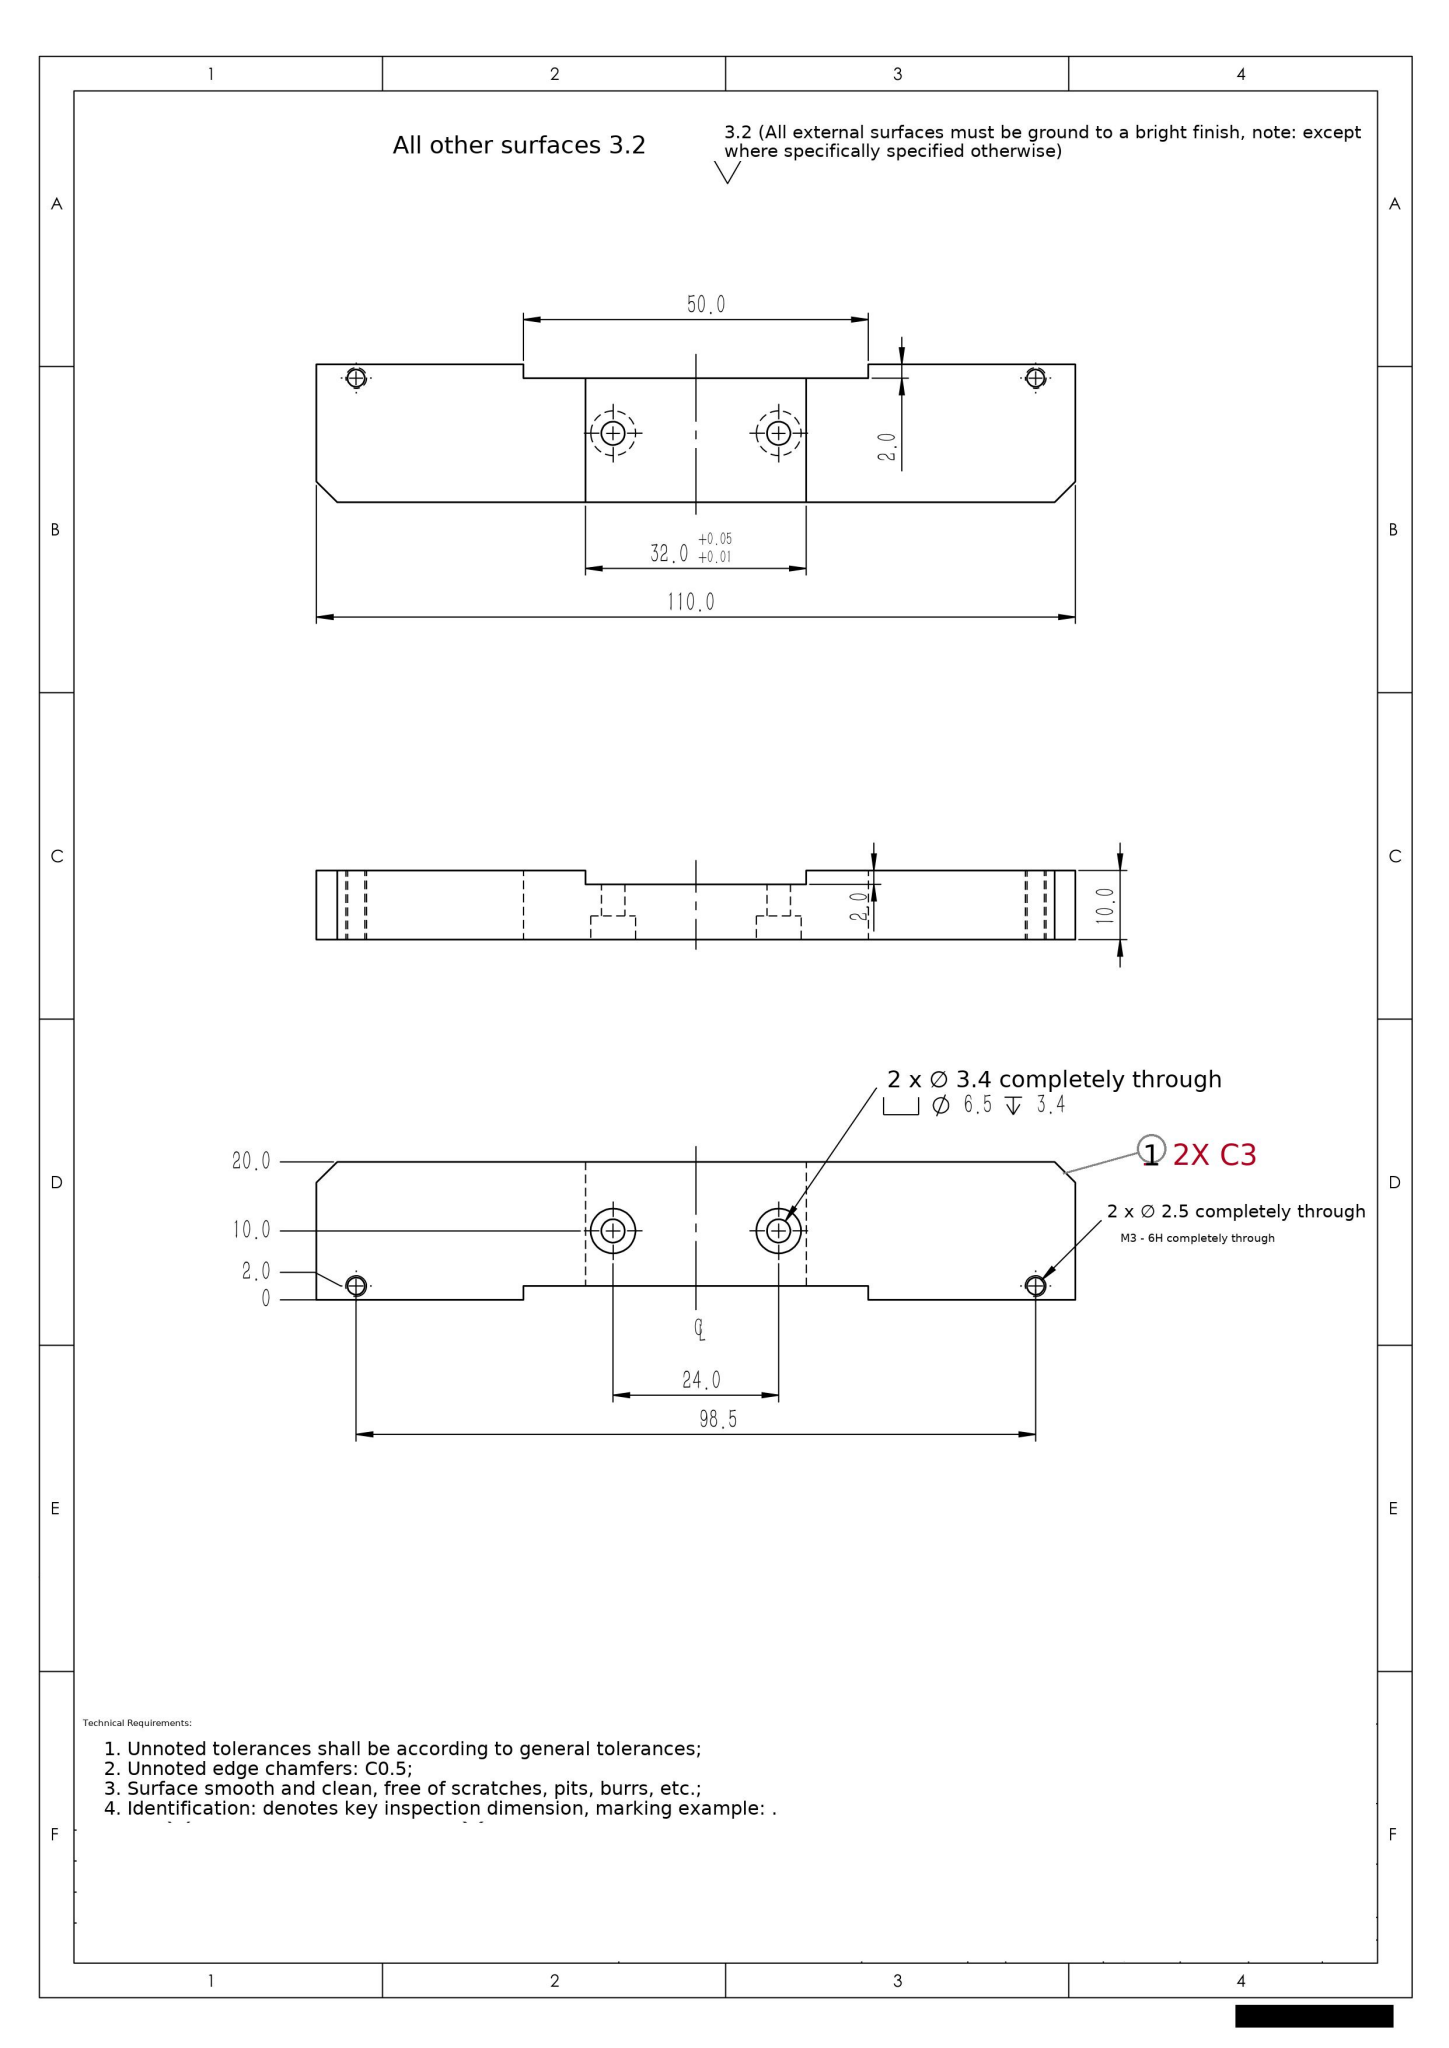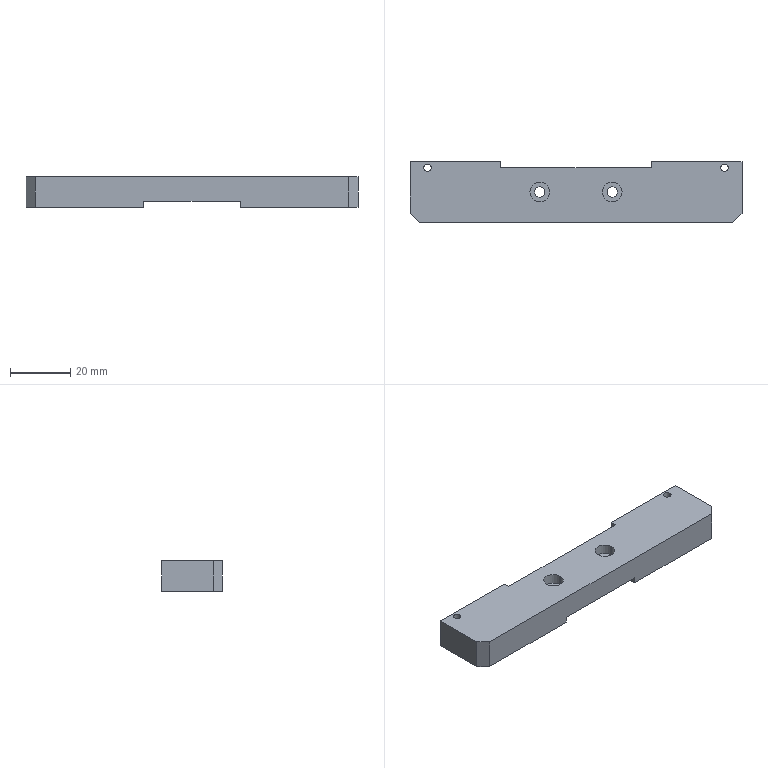Part | SolidWorks | mm | 1 solid | 30 faces | box 110 x 20 x 10 mm | volume 19351 mm3 | plane 18 | cylinder 12 | commonest cylinder face diameters 6.5 x4 3.4 x4 2.5 x4
build123d program:
from build123d import *

# Parameters (mm, degrees)
SKETCH1_W                                       = 110
SKETCH1_H                                       = 20
BOSS_EXTRUDE1_DEPTH                             = 5
M3_TAPPED_HOLE1_D                               = 2.5
M3_HEX_SOCKET_HEAD_CAP_SCREW_CBORE1_D           = 3.4
M3_HEX_SOCKET_HEAD_CAP_SCREW_CBORE1_CBORE_D     = 6.5
M3_HEX_SOCKET_HEAD_CAP_SCREW_CBORE1_CBORE_DEPTH = 3.4
SKETCH17_W                                      = 32
SKETCH17_H                                      = 18.5
CUT_EXTRUDE2_DEPTH                              = 2
SKETCH18_W                                      = 50
SKETCH18_H                                      = 2
CUT_EXTRUDE3_DEPTH                              = 57.789
CHAMFER1_SIZE                                   = 3


with BuildPart() as part:
    # Sketch1 → Boss-Extrude1 (new, symmetric)
    with BuildSketch(Plane.XY):
        Rectangle(SKETCH1_W, SKETCH1_H)
    extrude(amount=BOSS_EXTRUDE1_DEPTH, both=True)

    # M3 Tapped Hole1 (through all)
    with Locations(Plane.XY.offset(5)):
        with Locations((-49.25, 8), (49.25, 8)):
            Hole(M3_TAPPED_HOLE1_D / 2)

    # M3 Hex Socket Head Cap Screw CBORE1 (through all)
    with Locations(Plane.XY.offset(5)):
        with Locations((-12, 0), (12, 0)):
            CounterBoreHole(M3_HEX_SOCKET_HEAD_CAP_SCREW_CBORE1_D / 2, M3_HEX_SOCKET_HEAD_CAP_SCREW_CBORE1_CBORE_D / 2, M3_HEX_SOCKET_HEAD_CAP_SCREW_CBORE1_CBORE_DEPTH)

    # Sketch17 → Cut-Extrude2 (cut)
    with BuildSketch(Plane(origin=(0, 0, -5), x_dir=(-1, 0, 0), z_dir=(0, 0, -1))):
        with Locations((0, -0.75)):
            Rectangle(SKETCH17_W, SKETCH17_H)
    extrude(amount=-CUT_EXTRUDE2_DEPTH, mode=Mode.SUBTRACT)

    # Sketch18 → Cut-Extrude3 (cut, through all)
    with BuildSketch(Plane(origin=(0, 0, -5), x_dir=(-1, 0, 0), z_dir=(0, 0, -1))):
        with Locations((0, 9)):
            Rectangle(SKETCH18_W, SKETCH18_H)
    extrude(amount=-CUT_EXTRUDE3_DEPTH, mode=Mode.SUBTRACT)

    # Chamfer1
    chamfer1_edges = [part.edges().sort_by_distance(p)[0] for p in [
        (55, -10, 0),
        (-55, -10, 0),
    ]]
    chamfer(chamfer1_edges, length=CHAMFER1_SIZE)


solid = part.part
STEP:
#1=CARTESIAN_POINT('',(-15.25,0.,1.6));
#2=VERTEX_POINT('',#1);
#3=CARTESIAN_POINT('',(-8.75,0.,1.6));
#4=VERTEX_POINT('',#3);
#5=CARTESIAN_POINT('',(-12.,0.,1.6));
#6=DIRECTION('',(0.,0.,1.));
#7=DIRECTION('',(1.,0.,0.));
#8=AXIS2_PLACEMENT_3D('',#5,#6,#7);
#9=CIRCLE('',#8,3.25);
#10=EDGE_CURVE('',#2,#4,#9,.T.);
#11=ORIENTED_EDGE('',*,*,#10,.F.);
#12=CARTESIAN_POINT('',(-15.25,0.,5.));
#13=VERTEX_POINT('',#12);
#14=CARTESIAN_POINT('',(-15.25,0.,5.));
#15=DIRECTION('',(0.,0.,1.));
#16=VECTOR('',#15,1000.);
#17=LINE('',#14,#16);
#18=EDGE_CURVE('',#2,#13,#17,.T.);
#19=ORIENTED_EDGE('',*,*,#18,.T.);
#20=CARTESIAN_POINT('',(-8.75,0.,5.));
#21=VERTEX_POINT('',#20);
#22=CARTESIAN_POINT('',(-12.,0.,5.));
#23=DIRECTION('',(0.,0.,1.));
#24=DIRECTION('',(1.,0.,0.));
#25=AXIS2_PLACEMENT_3D('',#22,#23,#24);
#26=CIRCLE('',#25,3.25);
#27=EDGE_CURVE('',#13,#21,#26,.T.);
#28=ORIENTED_EDGE('',*,*,#27,.T.);
#29=CARTESIAN_POINT('',(-8.75,0.,5.));
#30=DIRECTION('',(0.,0.,1.));
#31=VECTOR('',#30,1000.);
#32=LINE('',#29,#31);
#33=EDGE_CURVE('',#4,#21,#32,.T.);
#34=ORIENTED_EDGE('',*,*,#33,.F.);
#35=EDGE_LOOP('',(#11,#19,#28,#34));
#36=FACE_OUTER_BOUND('',#35,.T.);
#37=CARTESIAN_POINT('',(-12.,0.,5.));
#38=DIRECTION('',(0.,0.,1.));
#39=DIRECTION('',(1.,0.,0.));
#40=AXIS2_PLACEMENT_3D('',#37,#38,#39);
#41=CYLINDRICAL_SURFACE('',#40,3.25);
#42=ADVANCED_FACE('',(#36),#41,.F.);
#43=CARTESIAN_POINT('',(-10.3,0.,-3.));
#44=VERTEX_POINT('',#43);
#45=CARTESIAN_POINT('',(-13.7,0.,-3.));
#46=VERTEX_POINT('',#45);
#47=CARTESIAN_POINT('',(-12.,0.,-3.));
#48=DIRECTION('',(0.,0.,-1.));
#49=DIRECTION('',(1.,0.,0.));
#50=AXIS2_PLACEMENT_3D('',#47,#48,#49);
#51=CIRCLE('',#50,1.7);
#52=EDGE_CURVE('',#44,#46,#51,.T.);
#53=ORIENTED_EDGE('',*,*,#52,.T.);
#54=CARTESIAN_POINT('',(-13.7,0.,1.6));
#55=VERTEX_POINT('',#54);
#56=CARTESIAN_POINT('',(-13.7,0.,5.));
#57=DIRECTION('',(0.,0.,1.));
#58=VECTOR('',#57,1000.);
#59=LINE('',#56,#58);
#60=EDGE_CURVE('',#46,#55,#59,.T.);
#61=ORIENTED_EDGE('',*,*,#60,.T.);
#62=CARTESIAN_POINT('',(-10.3,0.,1.6));
#63=VERTEX_POINT('',#62);
#64=CARTESIAN_POINT('',(-12.,0.,1.6));
#65=DIRECTION('',(0.,0.,1.));
#66=DIRECTION('',(1.,0.,0.));
#67=AXIS2_PLACEMENT_3D('',#64,#65,#66);
#68=CIRCLE('',#67,1.7);
#69=EDGE_CURVE('',#55,#63,#68,.T.);
#70=ORIENTED_EDGE('',*,*,#69,.T.);
#71=CARTESIAN_POINT('',(-10.3,0.,5.));
#72=DIRECTION('',(0.,0.,1.));
#73=VECTOR('',#72,1000.);
#74=LINE('',#71,#73);
#75=EDGE_CURVE('',#44,#63,#74,.T.);
#76=ORIENTED_EDGE('',*,*,#75,.F.);
#77=EDGE_LOOP('',(#53,#61,#70,#76));
#78=FACE_OUTER_BOUND('',#77,.T.);
#79=CARTESIAN_POINT('',(-12.,0.,5.));
#80=DIRECTION('',(0.,0.,1.));
#81=DIRECTION('',(1.,0.,0.));
#82=AXIS2_PLACEMENT_3D('',#79,#80,#81);
#83=CYLINDRICAL_SURFACE('',#82,1.7);
#84=ADVANCED_FACE('',(#78),#83,.F.);
#85=CARTESIAN_POINT('',(8.75,0.,1.6));
#86=VERTEX_POINT('',#85);
#87=CARTESIAN_POINT('',(15.25,0.,1.6));
#88=VERTEX_POINT('',#87);
#89=CARTESIAN_POINT('',(12.,0.,1.6));
#90=DIRECTION('',(0.,0.,1.));
#91=DIRECTION('',(1.,0.,0.));
#92=AXIS2_PLACEMENT_3D('',#89,#90,#91);
#93=CIRCLE('',#92,3.25);
#94=EDGE_CURVE('',#86,#88,#93,.T.);
#95=ORIENTED_EDGE('',*,*,#94,.F.);
#96=CARTESIAN_POINT('',(8.75,0.,5.));
#97=VERTEX_POINT('',#96);
#98=CARTESIAN_POINT('',(8.75,0.,5.));
#99=DIRECTION('',(0.,0.,1.));
#100=VECTOR('',#99,1000.);
#101=LINE('',#98,#100);
#102=EDGE_CURVE('',#86,#97,#101,.T.);
#103=ORIENTED_EDGE('',*,*,#102,.T.);
#104=CARTESIAN_POINT('',(15.25,0.,5.));
#105=VERTEX_POINT('',#104);
#106=CARTESIAN_POINT('',(12.,0.,5.));
#107=DIRECTION('',(0.,0.,1.));
#108=DIRECTION('',(1.,0.,0.));
#109=AXIS2_PLACEMENT_3D('',#106,#107,#108);
#110=CIRCLE('',#109,3.25);
#111=EDGE_CURVE('',#97,#105,#110,.T.);
#112=ORIENTED_EDGE('',*,*,#111,.T.);
#113=CARTESIAN_POINT('',(15.25,0.,5.));
#114=DIRECTION('',(0.,0.,1.));
#115=VECTOR('',#114,1000.);
#116=LINE('',#113,#115);
#117=EDGE_CURVE('',#88,#105,#116,.T.);
#118=ORIENTED_EDGE('',*,*,#117,.F.);
#119=EDGE_LOOP('',(#95,#103,#112,#118));
#120=FACE_OUTER_BOUND('',#119,.T.);
#121=CARTESIAN_POINT('',(12.,0.,5.));
#122=DIRECTION('',(0.,0.,1.));
#123=DIRECTION('',(1.,0.,0.));
#124=AXIS2_PLACEMENT_3D('',#121,#122,#123);
#125=CYLINDRICAL_SURFACE('',#124,3.25);
#126=ADVANCED_FACE('',(#120),#125,.F.);
#127=CARTESIAN_POINT('',(13.7,0.,-3.));
#128=VERTEX_POINT('',#127);
#129=CARTESIAN_POINT('',(10.3,0.,-3.));
#130=VERTEX_POINT('',#129);
#131=CARTESIAN_POINT('',(12.,0.,-3.));
#132=DIRECTION('',(0.,0.,-1.));
#133=DIRECTION('',(1.,0.,0.));
#134=AXIS2_PLACEMENT_3D('',#131,#132,#133);
#135=CIRCLE('',#134,1.7);
#136=EDGE_CURVE('',#128,#130,#135,.T.);
#137=ORIENTED_EDGE('',*,*,#136,.T.);
#138=CARTESIAN_POINT('',(10.3,0.,1.6));
#139=VERTEX_POINT('',#138);
#140=CARTESIAN_POINT('',(10.3,0.,5.));
#141=DIRECTION('',(0.,0.,1.));
#142=VECTOR('',#141,1000.);
#143=LINE('',#140,#142);
#144=EDGE_CURVE('',#130,#139,#143,.T.);
#145=ORIENTED_EDGE('',*,*,#144,.T.);
#146=CARTESIAN_POINT('',(13.7,0.,1.6));
#147=VERTEX_POINT('',#146);
#148=CARTESIAN_POINT('',(12.,0.,1.6));
#149=DIRECTION('',(0.,0.,1.));
#150=DIRECTION('',(1.,0.,0.));
#151=AXIS2_PLACEMENT_3D('',#148,#149,#150);
#152=CIRCLE('',#151,1.7);
#153=EDGE_CURVE('',#139,#147,#152,.T.);
#154=ORIENTED_EDGE('',*,*,#153,.T.);
#155=CARTESIAN_POINT('',(13.7,0.,5.));
#156=DIRECTION('',(0.,0.,1.));
#157=VECTOR('',#156,1000.);
#158=LINE('',#155,#157);
#159=EDGE_CURVE('',#128,#147,#158,.T.);
#160=ORIENTED_EDGE('',*,*,#159,.F.);
#161=EDGE_LOOP('',(#137,#145,#154,#160));
#162=FACE_OUTER_BOUND('',#161,.T.);
#163=CARTESIAN_POINT('',(12.,0.,5.));
#164=DIRECTION('',(0.,0.,1.));
#165=DIRECTION('',(1.,0.,0.));
#166=AXIS2_PLACEMENT_3D('',#163,#164,#165);
#167=CYLINDRICAL_SURFACE('',#166,1.7);
#168=ADVANCED_FACE('',(#162),#167,.F.);
#169=CARTESIAN_POINT('',(-50.5,8.,-5.));
#170=VERTEX_POINT('',#169);
#171=CARTESIAN_POINT('',(-48.,8.,-5.));
#172=VERTEX_POINT('',#171);
#173=CARTESIAN_POINT('',(-49.25,8.,-5.));
#174=DIRECTION('',(0.,0.,1.));
#175=DIRECTION('',(1.,0.,0.));
#176=AXIS2_PLACEMENT_3D('',#173,#174,#175);
#177=CIRCLE('',#176,1.25);
#178=EDGE_CURVE('',#170,#172,#177,.T.);
#179=ORIENTED_EDGE('',*,*,#178,.F.);
#180=CARTESIAN_POINT('',(-50.5,8.,5.));
#181=VERTEX_POINT('',#180);
#182=CARTESIAN_POINT('',(-50.5,8.,5.));
#183=DIRECTION('',(0.,0.,1.));
#184=VECTOR('',#183,1000.);
#185=LINE('',#182,#184);
#186=EDGE_CURVE('',#170,#181,#185,.T.);
#187=ORIENTED_EDGE('',*,*,#186,.T.);
#188=CARTESIAN_POINT('',(-48.,8.,5.));
#189=VERTEX_POINT('',#188);
#190=CARTESIAN_POINT('',(-49.25,8.,5.));
#191=DIRECTION('',(0.,0.,1.));
#192=DIRECTION('',(1.,0.,0.));
#193=AXIS2_PLACEMENT_3D('',#190,#191,#192);
#194=CIRCLE('',#193,1.25);
#195=EDGE_CURVE('',#181,#189,#194,.T.);
#196=ORIENTED_EDGE('',*,*,#195,.T.);
#197=CARTESIAN_POINT('',(-48.,8.,5.));
#198=DIRECTION('',(0.,0.,1.));
#199=VECTOR('',#198,1000.);
#200=LINE('',#197,#199);
#201=EDGE_CURVE('',#172,#189,#200,.T.);
#202=ORIENTED_EDGE('',*,*,#201,.F.);
#203=EDGE_LOOP('',(#179,#187,#196,#202));
#204=FACE_OUTER_BOUND('',#203,.T.);
#205=CARTESIAN_POINT('',(-49.25,8.,5.));
#206=DIRECTION('',(0.,0.,1.));
#207=DIRECTION('',(1.,0.,0.));
#208=AXIS2_PLACEMENT_3D('',#205,#206,#207);
#209=CYLINDRICAL_SURFACE('',#208,1.25);
#210=ADVANCED_FACE('',(#204),#209,.F.);
#211=CARTESIAN_POINT('',(48.,8.,-5.));
#212=VERTEX_POINT('',#211);
#213=CARTESIAN_POINT('',(50.5,8.,-5.));
#214=VERTEX_POINT('',#213);
#215=CARTESIAN_POINT('',(49.25,8.,-5.));
#216=DIRECTION('',(0.,0.,1.));
#217=DIRECTION('',(1.,0.,0.));
#218=AXIS2_PLACEMENT_3D('',#215,#216,#217);
#219=CIRCLE('',#218,1.25);
#220=EDGE_CURVE('',#212,#214,#219,.T.);
#221=ORIENTED_EDGE('',*,*,#220,.F.);
#222=CARTESIAN_POINT('',(48.,8.,5.));
#223=VERTEX_POINT('',#222);
#224=CARTESIAN_POINT('',(48.,8.,5.));
#225=DIRECTION('',(0.,0.,1.));
#226=VECTOR('',#225,1000.);
#227=LINE('',#224,#226);
#228=EDGE_CURVE('',#212,#223,#227,.T.);
#229=ORIENTED_EDGE('',*,*,#228,.T.);
#230=CARTESIAN_POINT('',(50.5,8.,5.));
#231=VERTEX_POINT('',#230);
#232=CARTESIAN_POINT('',(49.25,8.,5.));
#233=DIRECTION('',(0.,0.,1.));
#234=DIRECTION('',(1.,0.,0.));
#235=AXIS2_PLACEMENT_3D('',#232,#233,#234);
#236=CIRCLE('',#235,1.25);
#237=EDGE_CURVE('',#223,#231,#236,.T.);
#238=ORIENTED_EDGE('',*,*,#237,.T.);
#239=CARTESIAN_POINT('',(50.5,8.,5.));
#240=DIRECTION('',(0.,0.,1.));
#241=VECTOR('',#240,1000.);
#242=LINE('',#239,#241);
#243=EDGE_CURVE('',#214,#231,#242,.T.);
#244=ORIENTED_EDGE('',*,*,#243,.F.);
#245=EDGE_LOOP('',(#221,#229,#238,#244));
#246=FACE_OUTER_BOUND('',#245,.T.);
#247=CARTESIAN_POINT('',(49.25,8.,5.));
#248=DIRECTION('',(0.,0.,1.));
#249=DIRECTION('',(1.,0.,0.));
#250=AXIS2_PLACEMENT_3D('',#247,#248,#249);
#251=CYLINDRICAL_SURFACE('',#250,1.25);
#252=ADVANCED_FACE('',(#246),#251,.F.);
#253=CARTESIAN_POINT('',(-25.,10.,5.));
#254=VERTEX_POINT('',#253);
#255=CARTESIAN_POINT('',(-55.,10.,5.));
#256=VERTEX_POINT('',#255);
#257=CARTESIAN_POINT('',(-55.,10.,5.));
#258=DIRECTION('',(-1.,0.,0.));
#259=VECTOR('',#258,1000.);
#260=LINE('',#257,#259);
#261=EDGE_CURVE('',#254,#256,#260,.T.);
#262=ORIENTED_EDGE('',*,*,#261,.F.);
#263=CARTESIAN_POINT('',(-25.,10.,-5.));
#264=VERTEX_POINT('',#263);
#265=CARTESIAN_POINT('',(-25.,10.,5.));
#266=DIRECTION('',(0.,0.,-1.));
#267=VECTOR('',#266,1000.);
#268=LINE('',#265,#267);
#269=EDGE_CURVE('',#254,#264,#268,.T.);
#270=ORIENTED_EDGE('',*,*,#269,.T.);
#271=CARTESIAN_POINT('',(-55.,10.,-5.));
#272=VERTEX_POINT('',#271);
#273=CARTESIAN_POINT('',(-55.,10.,-5.));
#274=DIRECTION('',(-1.,0.,0.));
#275=VECTOR('',#274,1000.);
#276=LINE('',#273,#275);
#277=EDGE_CURVE('',#264,#272,#276,.T.);
#278=ORIENTED_EDGE('',*,*,#277,.T.);
#279=CARTESIAN_POINT('',(-55.,10.,5.));
#280=DIRECTION('',(0.,0.,-1.));
#281=VECTOR('',#280,1000.);
#282=LINE('',#279,#281);
#283=EDGE_CURVE('',#256,#272,#282,.T.);
#284=ORIENTED_EDGE('',*,*,#283,.F.);
#285=EDGE_LOOP('',(#262,#270,#278,#284));
#286=FACE_OUTER_BOUND('',#285,.T.);
#287=CARTESIAN_POINT('',(-55.,10.,5.));
#288=DIRECTION('',(0.,-1.,0.));
#289=DIRECTION('',(0.,0.,-1.));
#290=AXIS2_PLACEMENT_3D('',#287,#288,#289);
#291=PLANE('',#290);
#292=ADVANCED_FACE('',(#286),#291,.F.);
#293=CARTESIAN_POINT('',(-52.,-10.,-5.));
#294=VERTEX_POINT('',#293);
#295=CARTESIAN_POINT('',(-16.,-10.,-5.));
#296=VERTEX_POINT('',#295);
#297=CARTESIAN_POINT('',(-55.,-10.,-5.));
#298=DIRECTION('',(1.,0.,0.));
#299=VECTOR('',#298,1000.);
#300=LINE('',#297,#299);
#301=EDGE_CURVE('',#294,#296,#300,.T.);
#302=ORIENTED_EDGE('',*,*,#301,.F.);
#303=CARTESIAN_POINT('',(-55.,-7.,-5.));
#304=VERTEX_POINT('',#303);
#305=CARTESIAN_POINT('',(-31.,-31.,-5.));
#306=DIRECTION('',(-0.7071,0.7071,0.));
#307=VECTOR('',#306,1000.);
#308=LINE('',#305,#307);
#309=EDGE_CURVE('',#294,#304,#308,.T.);
#310=ORIENTED_EDGE('',*,*,#309,.T.);
#311=CARTESIAN_POINT('',(-55.,-10.,-5.));
#312=DIRECTION('',(0.,-1.,0.));
#313=VECTOR('',#312,1000.);
#314=LINE('',#311,#313);
#315=EDGE_CURVE('',#272,#304,#314,.T.);
#316=ORIENTED_EDGE('',*,*,#315,.F.);
#317=ORIENTED_EDGE('',*,*,#277,.F.);
#318=CARTESIAN_POINT('',(-25.,8.,-5.));
#319=VERTEX_POINT('',#318);
#320=CARTESIAN_POINT('',(-25.,10.,-5.));
#321=DIRECTION('',(-0.,1.,0.));
#322=VECTOR('',#321,1000.);
#323=LINE('',#320,#322);
#324=EDGE_CURVE('',#319,#264,#323,.T.);
#325=ORIENTED_EDGE('',*,*,#324,.F.);
#326=CARTESIAN_POINT('',(-16.,8.,-5.));
#327=VERTEX_POINT('',#326);
#328=CARTESIAN_POINT('',(-25.,8.,-5.));
#329=DIRECTION('',(-1.,-0.,0.));
#330=VECTOR('',#329,1000.);
#331=LINE('',#328,#330);
#332=EDGE_CURVE('',#327,#319,#331,.T.);
#333=ORIENTED_EDGE('',*,*,#332,.F.);
#334=CARTESIAN_POINT('',(-16.,8.5,-5.));
#335=DIRECTION('',(0.,1.,0.));
#336=VECTOR('',#335,1000.);
#337=LINE('',#334,#336);
#338=EDGE_CURVE('',#296,#327,#337,.T.);
#339=ORIENTED_EDGE('',*,*,#338,.F.);
#340=EDGE_LOOP('',(#302,#310,#316,#317,#325,#333,#339));
#341=FACE_OUTER_BOUND('',#340,.T.);
#342=CARTESIAN_POINT('',(-49.25,8.,-5.));
#343=DIRECTION('',(0.,0.,1.));
#344=DIRECTION('',(1.,0.,0.));
#345=AXIS2_PLACEMENT_3D('',#342,#343,#344);
#346=CIRCLE('',#345,1.25);
#347=EDGE_CURVE('',#172,#170,#346,.T.);
#348=ORIENTED_EDGE('',*,*,#347,.T.);
#349=ORIENTED_EDGE('',*,*,#178,.T.);
#350=EDGE_LOOP('',(#348,#349));
#351=FACE_BOUND('',#350,.T.);
#352=CARTESIAN_POINT('',(0.,0.,-5.));
#353=DIRECTION('',(0.,0.,-1.));
#354=DIRECTION('',(-1.,0.,0.));
#355=AXIS2_PLACEMENT_3D('',#352,#353,#354);
#356=PLANE('',#355);
#357=ADVANCED_FACE('',(#341,#351),#356,.T.);
#358=CARTESIAN_POINT('',(55.,-7.,5.));
#359=VERTEX_POINT('',#358);
#360=CARTESIAN_POINT('',(55.,10.,5.));
#361=VERTEX_POINT('',#360);
#362=CARTESIAN_POINT('',(55.,-10.,5.));
#363=DIRECTION('',(0.,1.,0.));
#364=VECTOR('',#363,1000.);
#365=LINE('',#362,#364);
#366=EDGE_CURVE('',#359,#361,#365,.T.);
#367=ORIENTED_EDGE('',*,*,#366,.F.);
#368=CARTESIAN_POINT('',(55.,-7.,-5.));
#369=VERTEX_POINT('',#368);
#370=CARTESIAN_POINT('',(55.,-7.,5.));
#371=DIRECTION('',(0.,0.,-1.));
#372=VECTOR('',#371,1000.);
#373=LINE('',#370,#372);
#374=EDGE_CURVE('',#359,#369,#373,.T.);
#375=ORIENTED_EDGE('',*,*,#374,.T.);
#376=CARTESIAN_POINT('',(55.,10.,-5.));
#377=VERTEX_POINT('',#376);
#378=CARTESIAN_POINT('',(55.,-10.,-5.));
#379=DIRECTION('',(0.,1.,0.));
#380=VECTOR('',#379,1000.);
#381=LINE('',#378,#380);
#382=EDGE_CURVE('',#369,#377,#381,.T.);
#383=ORIENTED_EDGE('',*,*,#382,.T.);
#384=CARTESIAN_POINT('',(55.,10.,5.));
#385=DIRECTION('',(0.,0.,-1.));
#386=VECTOR('',#385,1000.);
#387=LINE('',#384,#386);
#388=EDGE_CURVE('',#361,#377,#387,.T.);
#389=ORIENTED_EDGE('',*,*,#388,.F.);
#390=EDGE_LOOP('',(#367,#375,#383,#389));
#391=FACE_OUTER_BOUND('',#390,.T.);
#392=CARTESIAN_POINT('',(55.,-10.,5.));
#393=DIRECTION('',(-1.,0.,0.));
#394=DIRECTION('',(0.,0.,1.));
#395=AXIS2_PLACEMENT_3D('',#392,#393,#394);
#396=PLANE('',#395);
#397=ADVANCED_FACE('',(#391),#396,.F.);
#398=CARTESIAN_POINT('',(25.,10.,-5.));
#399=VERTEX_POINT('',#398);
#400=CARTESIAN_POINT('',(-55.,10.,-5.));
#401=DIRECTION('',(-1.,0.,0.));
#402=VECTOR('',#401,1000.);
#403=LINE('',#400,#402);
#404=EDGE_CURVE('',#377,#399,#403,.T.);
#405=ORIENTED_EDGE('',*,*,#404,.T.);
#406=CARTESIAN_POINT('',(25.,10.,5.));
#407=VERTEX_POINT('',#406);
#408=CARTESIAN_POINT('',(25.,10.,5.));
#409=DIRECTION('',(0.,0.,-1.));
#410=VECTOR('',#409,1000.);
#411=LINE('',#408,#410);
#412=EDGE_CURVE('',#407,#399,#411,.T.);
#413=ORIENTED_EDGE('',*,*,#412,.F.);
#414=CARTESIAN_POINT('',(-55.,10.,5.));
#415=DIRECTION('',(-1.,0.,0.));
#416=VECTOR('',#415,1000.);
#417=LINE('',#414,#416);
#418=EDGE_CURVE('',#361,#407,#417,.T.);
#419=ORIENTED_EDGE('',*,*,#418,.F.);
#420=ORIENTED_EDGE('',*,*,#388,.T.);
#421=EDGE_LOOP('',(#405,#413,#419,#420));
#422=FACE_OUTER_BOUND('',#421,.T.);
#423=CARTESIAN_POINT('',(-55.,10.,5.));
#424=DIRECTION('',(0.,-1.,0.));
#425=DIRECTION('',(0.,0.,-1.));
#426=AXIS2_PLACEMENT_3D('',#423,#424,#425);
#427=PLANE('',#426);
#428=ADVANCED_FACE('',(#422),#427,.F.);
#429=ORIENTED_EDGE('',*,*,#315,.T.);
#430=CARTESIAN_POINT('',(-55.,-7.,5.));
#431=VERTEX_POINT('',#430);
#432=CARTESIAN_POINT('',(-55.,-7.,5.));
#433=DIRECTION('',(0.,0.,1.));
#434=VECTOR('',#433,1000.);
#435=LINE('',#432,#434);
#436=EDGE_CURVE('',#304,#431,#435,.T.);
#437=ORIENTED_EDGE('',*,*,#436,.T.);
#438=CARTESIAN_POINT('',(-55.,-10.,5.));
#439=DIRECTION('',(0.,-1.,0.));
#440=VECTOR('',#439,1000.);
#441=LINE('',#438,#440);
#442=EDGE_CURVE('',#256,#431,#441,.T.);
#443=ORIENTED_EDGE('',*,*,#442,.F.);
#444=ORIENTED_EDGE('',*,*,#283,.T.);
#445=EDGE_LOOP('',(#429,#437,#443,#444));
#446=FACE_OUTER_BOUND('',#445,.T.);
#447=CARTESIAN_POINT('',(-55.,-10.,5.));
#448=DIRECTION('',(1.,0.,0.));
#449=DIRECTION('',(0.,0.,-1.));
#450=AXIS2_PLACEMENT_3D('',#447,#448,#449);
#451=PLANE('',#450);
#452=ADVANCED_FACE('',(#446),#451,.F.);
#453=CARTESIAN_POINT('',(16.,-10.,-5.));
#454=VERTEX_POINT('',#453);
#455=CARTESIAN_POINT('',(52.,-10.,-5.));
#456=VERTEX_POINT('',#455);
#457=CARTESIAN_POINT('',(-55.,-10.,-5.));
#458=DIRECTION('',(1.,0.,0.));
#459=VECTOR('',#458,1000.);
#460=LINE('',#457,#459);
#461=EDGE_CURVE('',#454,#456,#460,.T.);
#462=ORIENTED_EDGE('',*,*,#461,.T.);
#463=CARTESIAN_POINT('',(52.,-10.,5.));
#464=VERTEX_POINT('',#463);
#465=CARTESIAN_POINT('',(52.,-10.,5.));
#466=DIRECTION('',(0.,0.,1.));
#467=VECTOR('',#466,1000.);
#468=LINE('',#465,#467);
#469=EDGE_CURVE('',#456,#464,#468,.T.);
#470=ORIENTED_EDGE('',*,*,#469,.T.);
#471=CARTESIAN_POINT('',(-52.,-10.,5.));
#472=VERTEX_POINT('',#471);
#473=CARTESIAN_POINT('',(-55.,-10.,5.));
#474=DIRECTION('',(1.,0.,0.));
#475=VECTOR('',#474,1000.);
#476=LINE('',#473,#475);
#477=EDGE_CURVE('',#472,#464,#476,.T.);
#478=ORIENTED_EDGE('',*,*,#477,.F.);
#479=CARTESIAN_POINT('',(-52.,-10.,5.));
#480=DIRECTION('',(0.,0.,-1.));
#481=VECTOR('',#480,1000.);
#482=LINE('',#479,#481);
#483=EDGE_CURVE('',#472,#294,#482,.T.);
#484=ORIENTED_EDGE('',*,*,#483,.T.);
#485=ORIENTED_EDGE('',*,*,#301,.T.);
#486=CARTESIAN_POINT('',(-16.,-10.,-3.));
#487=VERTEX_POINT('',#486);
#488=CARTESIAN_POINT('',(-16.,-10.,-3.));
#489=DIRECTION('',(0.,0.,-1.));
#490=VECTOR('',#489,1000.);
#491=LINE('',#488,#490);
#492=EDGE_CURVE('',#487,#296,#491,.T.);
#493=ORIENTED_EDGE('',*,*,#492,.F.);
#494=CARTESIAN_POINT('',(16.,-10.,-3.));
#495=VERTEX_POINT('',#494);
#496=CARTESIAN_POINT('',(-16.,-10.,-3.));
#497=DIRECTION('',(-1.,-0.,0.));
#498=VECTOR('',#497,1000.);
#499=LINE('',#496,#498);
#500=EDGE_CURVE('',#495,#487,#499,.T.);
#501=ORIENTED_EDGE('',*,*,#500,.F.);
#502=CARTESIAN_POINT('',(16.,-10.,-3.));
#503=DIRECTION('',(0.,0.,-1.));
#504=VECTOR('',#503,1000.);
#505=LINE('',#502,#504);
#506=EDGE_CURVE('',#495,#454,#505,.T.);
#507=ORIENTED_EDGE('',*,*,#506,.T.);
#508=EDGE_LOOP('',(#462,#470,#478,#484,#485,#493,#501,#507));
#509=FACE_OUTER_BOUND('',#508,.T.);
#510=CARTESIAN_POINT('',(-55.,-10.,5.));
#511=DIRECTION('',(0.,1.,0.));
#512=DIRECTION('',(0.,0.,1.));
#513=AXIS2_PLACEMENT_3D('',#510,#511,#512);
#514=PLANE('',#513);
#515=ADVANCED_FACE('',(#509),#514,.F.);
#516=CARTESIAN_POINT('',(-12.,0.,5.));
#517=DIRECTION('',(0.,0.,1.));
#518=DIRECTION('',(1.,0.,0.));
#519=AXIS2_PLACEMENT_3D('',#516,#517,#518);
#520=CIRCLE('',#519,3.25);
#521=EDGE_CURVE('',#21,#13,#520,.T.);
#522=ORIENTED_EDGE('',*,*,#521,.F.);
#523=ORIENTED_EDGE('',*,*,#27,.F.);
#524=EDGE_LOOP('',(#522,#523));
#525=FACE_BOUND('',#524,.T.);
#526=CARTESIAN_POINT('',(12.,0.,5.));
#527=DIRECTION('',(0.,0.,1.));
#528=DIRECTION('',(1.,0.,0.));
#529=AXIS2_PLACEMENT_3D('',#526,#527,#528);
#530=CIRCLE('',#529,3.25);
#531=EDGE_CURVE('',#105,#97,#530,.T.);
#532=ORIENTED_EDGE('',*,*,#531,.F.);
#533=ORIENTED_EDGE('',*,*,#111,.F.);
#534=EDGE_LOOP('',(#532,#533));
#535=FACE_BOUND('',#534,.T.);
#536=CARTESIAN_POINT('',(-49.25,8.,5.));
#537=DIRECTION('',(0.,0.,1.));
#538=DIRECTION('',(1.,0.,0.));
#539=AXIS2_PLACEMENT_3D('',#536,#537,#538);
#540=CIRCLE('',#539,1.25);
#541=EDGE_CURVE('',#189,#181,#540,.T.);
#542=ORIENTED_EDGE('',*,*,#541,.F.);
#543=ORIENTED_EDGE('',*,*,#195,.F.);
#544=EDGE_LOOP('',(#542,#543));
#545=FACE_BOUND('',#544,.T.);
#546=CARTESIAN_POINT('',(49.25,8.,5.));
#547=DIRECTION('',(0.,0.,1.));
#548=DIRECTION('',(1.,0.,0.));
#549=AXIS2_PLACEMENT_3D('',#546,#547,#548);
#550=CIRCLE('',#549,1.25);
#551=EDGE_CURVE('',#231,#223,#550,.T.);
#552=ORIENTED_EDGE('',*,*,#551,.F.);
#553=ORIENTED_EDGE('',*,*,#237,.F.);
#554=EDGE_LOOP('',(#552,#553));
#555=FACE_BOUND('',#554,.T.);
#556=ORIENTED_EDGE('',*,*,#477,.T.);
#557=CARTESIAN_POINT('',(55.,-7.,5.));
#558=DIRECTION('',(0.7071,0.7071,0.));
#559=VECTOR('',#558,1000.);
#560=LINE('',#557,#559);
#561=EDGE_CURVE('',#464,#359,#560,.T.);
#562=ORIENTED_EDGE('',*,*,#561,.T.);
#563=ORIENTED_EDGE('',*,*,#366,.T.);
#564=ORIENTED_EDGE('',*,*,#418,.T.);
#565=CARTESIAN_POINT('',(25.,8.,5.));
#566=VERTEX_POINT('',#565);
#567=CARTESIAN_POINT('',(25.,10.,5.));
#568=DIRECTION('',(0.,-1.,0.));
#569=VECTOR('',#568,1000.);
#570=LINE('',#567,#569);
#571=EDGE_CURVE('',#407,#566,#570,.T.);
#572=ORIENTED_EDGE('',*,*,#571,.T.);
#573=CARTESIAN_POINT('',(-25.,8.,5.));
#574=VERTEX_POINT('',#573);
#575=CARTESIAN_POINT('',(-25.,8.,5.));
#576=DIRECTION('',(-1.,-0.,0.));
#577=VECTOR('',#576,1000.);
#578=LINE('',#575,#577);
#579=EDGE_CURVE('',#566,#574,#578,.T.);
#580=ORIENTED_EDGE('',*,*,#579,.T.);
#581=CARTESIAN_POINT('',(-25.,10.,5.));
#582=DIRECTION('',(-0.,1.,0.));
#583=VECTOR('',#582,1000.);
#584=LINE('',#581,#583);
#585=EDGE_CURVE('',#574,#254,#584,.T.);
#586=ORIENTED_EDGE('',*,*,#585,.T.);
#587=ORIENTED_EDGE('',*,*,#261,.T.);
#588=ORIENTED_EDGE('',*,*,#442,.T.);
#589=CARTESIAN_POINT('',(-52.,-10.,5.));
#590=DIRECTION('',(0.7071,-0.7071,0.));
#591=VECTOR('',#590,1000.);
#592=LINE('',#589,#591);
#593=EDGE_CURVE('',#431,#472,#592,.T.);
#594=ORIENTED_EDGE('',*,*,#593,.T.);
#595=EDGE_LOOP('',(#556,#562,#563,#564,#572,#580,#586,#587,#588,#594));
#596=FACE_OUTER_BOUND('',#595,.T.);
#597=CARTESIAN_POINT('',(0.,0.,5.));
#598=DIRECTION('',(0.,0.,-1.));
#599=DIRECTION('',(-1.,0.,0.));
#600=AXIS2_PLACEMENT_3D('',#597,#598,#599);
#601=PLANE('',#600);
#602=ADVANCED_FACE('',(#525,#535,#545,#555,#596),#601,.F.);
#603=ORIENTED_EDGE('',*,*,#382,.F.);
#604=CARTESIAN_POINT('',(31.,-31.,-5.));
#605=DIRECTION('',(-0.7071,-0.7071,0.));
#606=VECTOR('',#605,1000.);
#607=LINE('',#604,#606);
#608=EDGE_CURVE('',#369,#456,#607,.T.);
#609=ORIENTED_EDGE('',*,*,#608,.T.);
#610=ORIENTED_EDGE('',*,*,#461,.F.);
#611=CARTESIAN_POINT('',(16.,8.,-5.));
#612=VERTEX_POINT('',#611);
#613=CARTESIAN_POINT('',(16.,8.5,-5.));
#614=DIRECTION('',(0.,-1.,0.));
#615=VECTOR('',#614,1000.);
#616=LINE('',#613,#615);
#617=EDGE_CURVE('',#612,#454,#616,.T.);
#618=ORIENTED_EDGE('',*,*,#617,.F.);
#619=CARTESIAN_POINT('',(25.,8.,-5.));
#620=VERTEX_POINT('',#619);
#621=CARTESIAN_POINT('',(-25.,8.,-5.));
#622=DIRECTION('',(-1.,-0.,0.));
#623=VECTOR('',#622,1000.);
#624=LINE('',#621,#623);
#625=EDGE_CURVE('',#620,#612,#624,.T.);
#626=ORIENTED_EDGE('',*,*,#625,.F.);
#627=CARTESIAN_POINT('',(25.,10.,-5.));
#628=DIRECTION('',(0.,-1.,0.));
#629=VECTOR('',#628,1000.);
#630=LINE('',#627,#629);
#631=EDGE_CURVE('',#399,#620,#630,.T.);
#632=ORIENTED_EDGE('',*,*,#631,.F.);
#633=ORIENTED_EDGE('',*,*,#404,.F.);
#634=EDGE_LOOP('',(#603,#609,#610,#618,#626,#632,#633));
#635=FACE_OUTER_BOUND('',#634,.T.);
#636=CARTESIAN_POINT('',(49.25,8.,-5.));
#637=DIRECTION('',(0.,0.,1.));
#638=DIRECTION('',(1.,0.,0.));
#639=AXIS2_PLACEMENT_3D('',#636,#637,#638);
#640=CIRCLE('',#639,1.25);
#641=EDGE_CURVE('',#214,#212,#640,.T.);
#642=ORIENTED_EDGE('',*,*,#641,.T.);
#643=ORIENTED_EDGE('',*,*,#220,.T.);
#644=EDGE_LOOP('',(#642,#643));
#645=FACE_BOUND('',#644,.T.);
#646=CARTESIAN_POINT('',(0.,0.,-5.));
#647=DIRECTION('',(0.,0.,-1.));
#648=DIRECTION('',(-1.,0.,0.));
#649=AXIS2_PLACEMENT_3D('',#646,#647,#648);
#650=PLANE('',#649);
#651=ADVANCED_FACE('',(#635,#645),#650,.T.);
#652=ORIENTED_EDGE('',*,*,#228,.F.);
#653=ORIENTED_EDGE('',*,*,#641,.F.);
#654=ORIENTED_EDGE('',*,*,#243,.T.);
#655=ORIENTED_EDGE('',*,*,#551,.T.);
#656=EDGE_LOOP('',(#652,#653,#654,#655));
#657=FACE_OUTER_BOUND('',#656,.T.);
#658=CARTESIAN_POINT('',(49.25,8.,5.));
#659=DIRECTION('',(0.,0.,1.));
#660=DIRECTION('',(1.,0.,0.));
#661=AXIS2_PLACEMENT_3D('',#658,#659,#660);
#662=CYLINDRICAL_SURFACE('',#661,1.25);
#663=ADVANCED_FACE('',(#657),#662,.F.);
#664=ORIENTED_EDGE('',*,*,#186,.F.);
#665=ORIENTED_EDGE('',*,*,#347,.F.);
#666=ORIENTED_EDGE('',*,*,#201,.T.);
#667=ORIENTED_EDGE('',*,*,#541,.T.);
#668=EDGE_LOOP('',(#664,#665,#666,#667));
#669=FACE_OUTER_BOUND('',#668,.T.);
#670=CARTESIAN_POINT('',(-49.25,8.,5.));
#671=DIRECTION('',(0.,0.,1.));
#672=DIRECTION('',(1.,0.,0.));
#673=AXIS2_PLACEMENT_3D('',#670,#671,#672);
#674=CYLINDRICAL_SURFACE('',#673,1.25);
#675=ADVANCED_FACE('',(#669),#674,.F.);
#676=ORIENTED_EDGE('',*,*,#144,.F.);
#677=CARTESIAN_POINT('',(12.,0.,-3.));
#678=DIRECTION('',(0.,0.,-1.));
#679=DIRECTION('',(1.,0.,0.));
#680=AXIS2_PLACEMENT_3D('',#677,#678,#679);
#681=CIRCLE('',#680,1.7);
#682=EDGE_CURVE('',#130,#128,#681,.T.);
#683=ORIENTED_EDGE('',*,*,#682,.T.);
#684=ORIENTED_EDGE('',*,*,#159,.T.);
#685=CARTESIAN_POINT('',(12.,0.,1.6));
#686=DIRECTION('',(0.,0.,1.));
#687=DIRECTION('',(1.,0.,0.));
#688=AXIS2_PLACEMENT_3D('',#685,#686,#687);
#689=CIRCLE('',#688,1.7);
#690=EDGE_CURVE('',#147,#139,#689,.T.);
#691=ORIENTED_EDGE('',*,*,#690,.T.);
#692=EDGE_LOOP('',(#676,#683,#684,#691));
#693=FACE_OUTER_BOUND('',#692,.T.);
#694=CARTESIAN_POINT('',(12.,0.,5.));
#695=DIRECTION('',(0.,0.,1.));
#696=DIRECTION('',(1.,0.,0.));
#697=AXIS2_PLACEMENT_3D('',#694,#695,#696);
#698=CYLINDRICAL_SURFACE('',#697,1.7);
#699=ADVANCED_FACE('',(#693),#698,.F.);
#700=ORIENTED_EDGE('',*,*,#690,.F.);
#701=ORIENTED_EDGE('',*,*,#153,.F.);
#702=EDGE_LOOP('',(#700,#701));
#703=FACE_BOUND('',#702,.T.);
#704=CARTESIAN_POINT('',(12.,0.,1.6));
#705=DIRECTION('',(0.,0.,1.));
#706=DIRECTION('',(1.,0.,0.));
#707=AXIS2_PLACEMENT_3D('',#704,#705,#706);
#708=CIRCLE('',#707,3.25);
#709=EDGE_CURVE('',#88,#86,#708,.T.);
#710=ORIENTED_EDGE('',*,*,#709,.T.);
#711=ORIENTED_EDGE('',*,*,#94,.T.);
#712=EDGE_LOOP('',(#710,#711));
#713=FACE_OUTER_BOUND('',#712,.T.);
#714=CARTESIAN_POINT('',(13.7,0.,1.6));
#715=DIRECTION('',(0.,0.,-1.));
#716=DIRECTION('',(-1.,0.,0.));
#717=AXIS2_PLACEMENT_3D('',#714,#715,#716);
#718=PLANE('',#717);
#719=ADVANCED_FACE('',(#703,#713),#718,.F.);
#720=ORIENTED_EDGE('',*,*,#102,.F.);
#721=ORIENTED_EDGE('',*,*,#709,.F.);
#722=ORIENTED_EDGE('',*,*,#117,.T.);
#723=ORIENTED_EDGE('',*,*,#531,.T.);
#724=EDGE_LOOP('',(#720,#721,#722,#723));
#725=FACE_OUTER_BOUND('',#724,.T.);
#726=CARTESIAN_POINT('',(12.,0.,5.));
#727=DIRECTION('',(0.,0.,1.));
#728=DIRECTION('',(1.,0.,0.));
#729=AXIS2_PLACEMENT_3D('',#726,#727,#728);
#730=CYLINDRICAL_SURFACE('',#729,3.25);
#731=ADVANCED_FACE('',(#725),#730,.F.);
#732=ORIENTED_EDGE('',*,*,#60,.F.);
#733=CARTESIAN_POINT('',(-12.,0.,-3.));
#734=DIRECTION('',(0.,0.,-1.));
#735=DIRECTION('',(1.,0.,0.));
#736=AXIS2_PLACEMENT_3D('',#733,#734,#735);
#737=CIRCLE('',#736,1.7);
#738=EDGE_CURVE('',#46,#44,#737,.T.);
#739=ORIENTED_EDGE('',*,*,#738,.T.);
#740=ORIENTED_EDGE('',*,*,#75,.T.);
#741=CARTESIAN_POINT('',(-12.,0.,1.6));
#742=DIRECTION('',(0.,0.,1.));
#743=DIRECTION('',(1.,0.,0.));
#744=AXIS2_PLACEMENT_3D('',#741,#742,#743);
#745=CIRCLE('',#744,1.7);
#746=EDGE_CURVE('',#63,#55,#745,.T.);
#747=ORIENTED_EDGE('',*,*,#746,.T.);
#748=EDGE_LOOP('',(#732,#739,#740,#747));
#749=FACE_OUTER_BOUND('',#748,.T.);
#750=CARTESIAN_POINT('',(-12.,0.,5.));
#751=DIRECTION('',(0.,0.,1.));
#752=DIRECTION('',(1.,0.,0.));
#753=AXIS2_PLACEMENT_3D('',#750,#751,#752);
#754=CYLINDRICAL_SURFACE('',#753,1.7);
#755=ADVANCED_FACE('',(#749),#754,.F.);
#756=ORIENTED_EDGE('',*,*,#746,.F.);
#757=ORIENTED_EDGE('',*,*,#69,.F.);
#758=EDGE_LOOP('',(#756,#757));
#759=FACE_BOUND('',#758,.T.);
#760=CARTESIAN_POINT('',(-12.,0.,1.6));
#761=DIRECTION('',(0.,0.,1.));
#762=DIRECTION('',(1.,0.,0.));
#763=AXIS2_PLACEMENT_3D('',#760,#761,#762);
#764=CIRCLE('',#763,3.25);
#765=EDGE_CURVE('',#4,#2,#764,.T.);
#766=ORIENTED_EDGE('',*,*,#765,.T.);
#767=ORIENTED_EDGE('',*,*,#10,.T.);
#768=EDGE_LOOP('',(#766,#767));
#769=FACE_OUTER_BOUND('',#768,.T.);
#770=CARTESIAN_POINT('',(-10.3,0.,1.6));
#771=DIRECTION('',(0.,0.,-1.));
#772=DIRECTION('',(-1.,0.,0.));
#773=AXIS2_PLACEMENT_3D('',#770,#771,#772);
#774=PLANE('',#773);
#775=ADVANCED_FACE('',(#759,#769),#774,.F.);
#776=ORIENTED_EDGE('',*,*,#18,.F.);
#777=ORIENTED_EDGE('',*,*,#765,.F.);
#778=ORIENTED_EDGE('',*,*,#33,.T.);
#779=ORIENTED_EDGE('',*,*,#521,.T.);
#780=EDGE_LOOP('',(#776,#777,#778,#779));
#781=FACE_OUTER_BOUND('',#780,.T.);
#782=CARTESIAN_POINT('',(-12.,0.,5.));
#783=DIRECTION('',(0.,0.,1.));
#784=DIRECTION('',(1.,0.,0.));
#785=AXIS2_PLACEMENT_3D('',#782,#783,#784);
#786=CYLINDRICAL_SURFACE('',#785,3.25);
#787=ADVANCED_FACE('',(#781),#786,.F.);
#788=ORIENTED_EDGE('',*,*,#52,.F.);
#789=ORIENTED_EDGE('',*,*,#738,.F.);
#790=EDGE_LOOP('',(#788,#789));
#791=FACE_BOUND('',#790,.T.);
#792=CARTESIAN_POINT('',(-16.,8.,-3.));
#793=VERTEX_POINT('',#792);
#794=CARTESIAN_POINT('',(-16.,8.5,-3.));
#795=DIRECTION('',(0.,1.,0.));
#796=VECTOR('',#795,1000.);
#797=LINE('',#794,#796);
#798=EDGE_CURVE('',#487,#793,#797,.T.);
#799=ORIENTED_EDGE('',*,*,#798,.T.);
#800=CARTESIAN_POINT('',(16.,8.,-3.));
#801=VERTEX_POINT('',#800);
#802=CARTESIAN_POINT('',(-0.,8.,-3.));
#803=DIRECTION('',(1.,0.,0.));
#804=VECTOR('',#803,1000.);
#805=LINE('',#802,#804);
#806=EDGE_CURVE('',#793,#801,#805,.T.);
#807=ORIENTED_EDGE('',*,*,#806,.T.);
#808=CARTESIAN_POINT('',(16.,8.5,-3.));
#809=DIRECTION('',(0.,-1.,0.));
#810=VECTOR('',#809,1000.);
#811=LINE('',#808,#810);
#812=EDGE_CURVE('',#801,#495,#811,.T.);
#813=ORIENTED_EDGE('',*,*,#812,.T.);
#814=ORIENTED_EDGE('',*,*,#500,.T.);
#815=EDGE_LOOP('',(#799,#807,#813,#814));
#816=FACE_OUTER_BOUND('',#815,.T.);
#817=ORIENTED_EDGE('',*,*,#136,.F.);
#818=ORIENTED_EDGE('',*,*,#682,.F.);
#819=EDGE_LOOP('',(#817,#818));
#820=FACE_BOUND('',#819,.T.);
#821=CARTESIAN_POINT('',(0.,0.,-3.));
#822=DIRECTION('',(0.,0.,1.));
#823=DIRECTION('',(1.,0.,0.));
#824=AXIS2_PLACEMENT_3D('',#821,#822,#823);
#825=PLANE('',#824);
#826=ADVANCED_FACE('',(#791,#816,#820),#825,.F.);
#827=ORIENTED_EDGE('',*,*,#338,.T.);
#828=CARTESIAN_POINT('',(-16.,8.,-3.));
#829=DIRECTION('',(0.,0.,1.));
#830=VECTOR('',#829,1000.);
#831=LINE('',#828,#830);
#832=EDGE_CURVE('',#327,#793,#831,.T.);
#833=ORIENTED_EDGE('',*,*,#832,.T.);
#834=ORIENTED_EDGE('',*,*,#798,.F.);
#835=ORIENTED_EDGE('',*,*,#492,.T.);
#836=EDGE_LOOP('',(#827,#833,#834,#835));
#837=FACE_OUTER_BOUND('',#836,.T.);
#838=CARTESIAN_POINT('',(-16.,8.5,-3.));
#839=DIRECTION('',(-1.,0.,0.));
#840=DIRECTION('',(-0.,-1.,0.));
#841=AXIS2_PLACEMENT_3D('',#838,#839,#840);
#842=PLANE('',#841);
#843=ADVANCED_FACE('',(#837),#842,.F.);
#844=ORIENTED_EDGE('',*,*,#812,.F.);
#845=CARTESIAN_POINT('',(16.,8.,-3.));
#846=DIRECTION('',(0.,0.,-1.));
#847=VECTOR('',#846,1000.);
#848=LINE('',#845,#847);
#849=EDGE_CURVE('',#801,#612,#848,.T.);
#850=ORIENTED_EDGE('',*,*,#849,.T.);
#851=ORIENTED_EDGE('',*,*,#617,.T.);
#852=ORIENTED_EDGE('',*,*,#506,.F.);
#853=EDGE_LOOP('',(#844,#850,#851,#852));
#854=FACE_OUTER_BOUND('',#853,.T.);
#855=CARTESIAN_POINT('',(16.,8.5,-3.));
#856=DIRECTION('',(1.,0.,0.));
#857=DIRECTION('',(0.,0.,-1.));
#858=AXIS2_PLACEMENT_3D('',#855,#856,#857);
#859=PLANE('',#858);
#860=ADVANCED_FACE('',(#854),#859,.F.);
#861=ORIENTED_EDGE('',*,*,#332,.T.);
#862=CARTESIAN_POINT('',(-25.,8.,5.));
#863=DIRECTION('',(0.,0.,-1.));
#864=VECTOR('',#863,1000.);
#865=LINE('',#862,#864);
#866=EDGE_CURVE('',#574,#319,#865,.T.);
#867=ORIENTED_EDGE('',*,*,#866,.F.);
#868=ORIENTED_EDGE('',*,*,#579,.F.);
#869=CARTESIAN_POINT('',(25.,8.,5.));
#870=DIRECTION('',(0.,0.,-1.));
#871=VECTOR('',#870,1000.);
#872=LINE('',#869,#871);
#873=EDGE_CURVE('',#566,#620,#872,.T.);
#874=ORIENTED_EDGE('',*,*,#873,.T.);
#875=ORIENTED_EDGE('',*,*,#625,.T.);
#876=ORIENTED_EDGE('',*,*,#849,.F.);
#877=ORIENTED_EDGE('',*,*,#806,.F.);
#878=ORIENTED_EDGE('',*,*,#832,.F.);
#879=EDGE_LOOP('',(#861,#867,#868,#874,#875,#876,#877,#878));
#880=FACE_OUTER_BOUND('',#879,.T.);
#881=CARTESIAN_POINT('',(-25.,8.,5.));
#882=DIRECTION('',(0.,-1.,0.));
#883=DIRECTION('',(1.,0.,0.));
#884=AXIS2_PLACEMENT_3D('',#881,#882,#883);
#885=PLANE('',#884);
#886=ADVANCED_FACE('',(#880),#885,.F.);
#887=ORIENTED_EDGE('',*,*,#324,.T.);
#888=ORIENTED_EDGE('',*,*,#269,.F.);
#889=ORIENTED_EDGE('',*,*,#585,.F.);
#890=ORIENTED_EDGE('',*,*,#866,.T.);
#891=EDGE_LOOP('',(#887,#888,#889,#890));
#892=FACE_OUTER_BOUND('',#891,.T.);
#893=CARTESIAN_POINT('',(-25.,10.,5.));
#894=DIRECTION('',(-1.,-0.,0.));
#895=DIRECTION('',(0.,-1.,0.));
#896=AXIS2_PLACEMENT_3D('',#893,#894,#895);
#897=PLANE('',#896);
#898=ADVANCED_FACE('',(#892),#897,.F.);
#899=ORIENTED_EDGE('',*,*,#631,.T.);
#900=ORIENTED_EDGE('',*,*,#873,.F.);
#901=ORIENTED_EDGE('',*,*,#571,.F.);
#902=ORIENTED_EDGE('',*,*,#412,.T.);
#903=EDGE_LOOP('',(#899,#900,#901,#902));
#904=FACE_OUTER_BOUND('',#903,.T.);
#905=CARTESIAN_POINT('',(25.,10.,5.));
#906=DIRECTION('',(1.,0.,0.));
#907=DIRECTION('',(0.,0.,-1.));
#908=AXIS2_PLACEMENT_3D('',#905,#906,#907);
#909=PLANE('',#908);
#910=ADVANCED_FACE('',(#904),#909,.F.);
#911=ORIENTED_EDGE('',*,*,#561,.F.);
#912=ORIENTED_EDGE('',*,*,#469,.F.);
#913=ORIENTED_EDGE('',*,*,#608,.F.);
#914=ORIENTED_EDGE('',*,*,#374,.F.);
#915=EDGE_LOOP('',(#911,#912,#913,#914));
#916=FACE_OUTER_BOUND('',#915,.T.);
#917=CARTESIAN_POINT('',(55.,-7.,5.));
#918=DIRECTION('',(-0.7071,0.7071,0.));
#919=DIRECTION('',(0.,0.,-1.));
#920=AXIS2_PLACEMENT_3D('',#917,#918,#919);
#921=PLANE('',#920);
#922=ADVANCED_FACE('',(#916),#921,.F.);
#923=ORIENTED_EDGE('',*,*,#593,.F.);
#924=ORIENTED_EDGE('',*,*,#436,.F.);
#925=ORIENTED_EDGE('',*,*,#309,.F.);
#926=ORIENTED_EDGE('',*,*,#483,.F.);
#927=EDGE_LOOP('',(#923,#924,#925,#926));
#928=FACE_OUTER_BOUND('',#927,.T.);
#929=CARTESIAN_POINT('',(-52.,-10.,5.));
#930=DIRECTION('',(0.7071,0.7071,0.));
#931=DIRECTION('',(0.,0.,-1.));
#932=AXIS2_PLACEMENT_3D('',#929,#930,#931);
#933=PLANE('',#932);
#934=ADVANCED_FACE('',(#928),#933,.F.);
#935=CLOSED_SHELL('',(#42,#84,#126,#168,#210,#252,#292,#357,#397,#428,#452,#515,#602,#651,#663,#675,#699,#719,#731,#755,#775,#787,#826,#843,#860,#886,#898,#910,#922,#934));
#936=MANIFOLD_SOLID_BREP('',#935);
#937=CARTESIAN_POINT('',(0.,0.,0.));
#938=DIRECTION('',(0.,0.,1.));
#939=DIRECTION('',(1.,0.,0.));
#940=AXIS2_PLACEMENT_3D('',#937,#938,#939);
#941=(LENGTH_UNIT()NAMED_UNIT(*)SI_UNIT(.MILLI.,.METRE.));
#942=UNCERTAINTY_MEASURE_WITH_UNIT(LENGTH_MEASURE(0.00001),#941,'','');
#943=(NAMED_UNIT(*)PLANE_ANGLE_UNIT()SI_UNIT($,.RADIAN.));
#944=(NAMED_UNIT(*)SI_UNIT($,.STERADIAN.)SOLID_ANGLE_UNIT());
#945=(GEOMETRIC_REPRESENTATION_CONTEXT(3)GLOBAL_UNCERTAINTY_ASSIGNED_CONTEXT((#942))GLOBAL_UNIT_ASSIGNED_CONTEXT((#941,#943,#944))REPRESENTATION_CONTEXT('',''));
#946=ADVANCED_BREP_SHAPE_REPRESENTATION('',(#936,#940),#945);